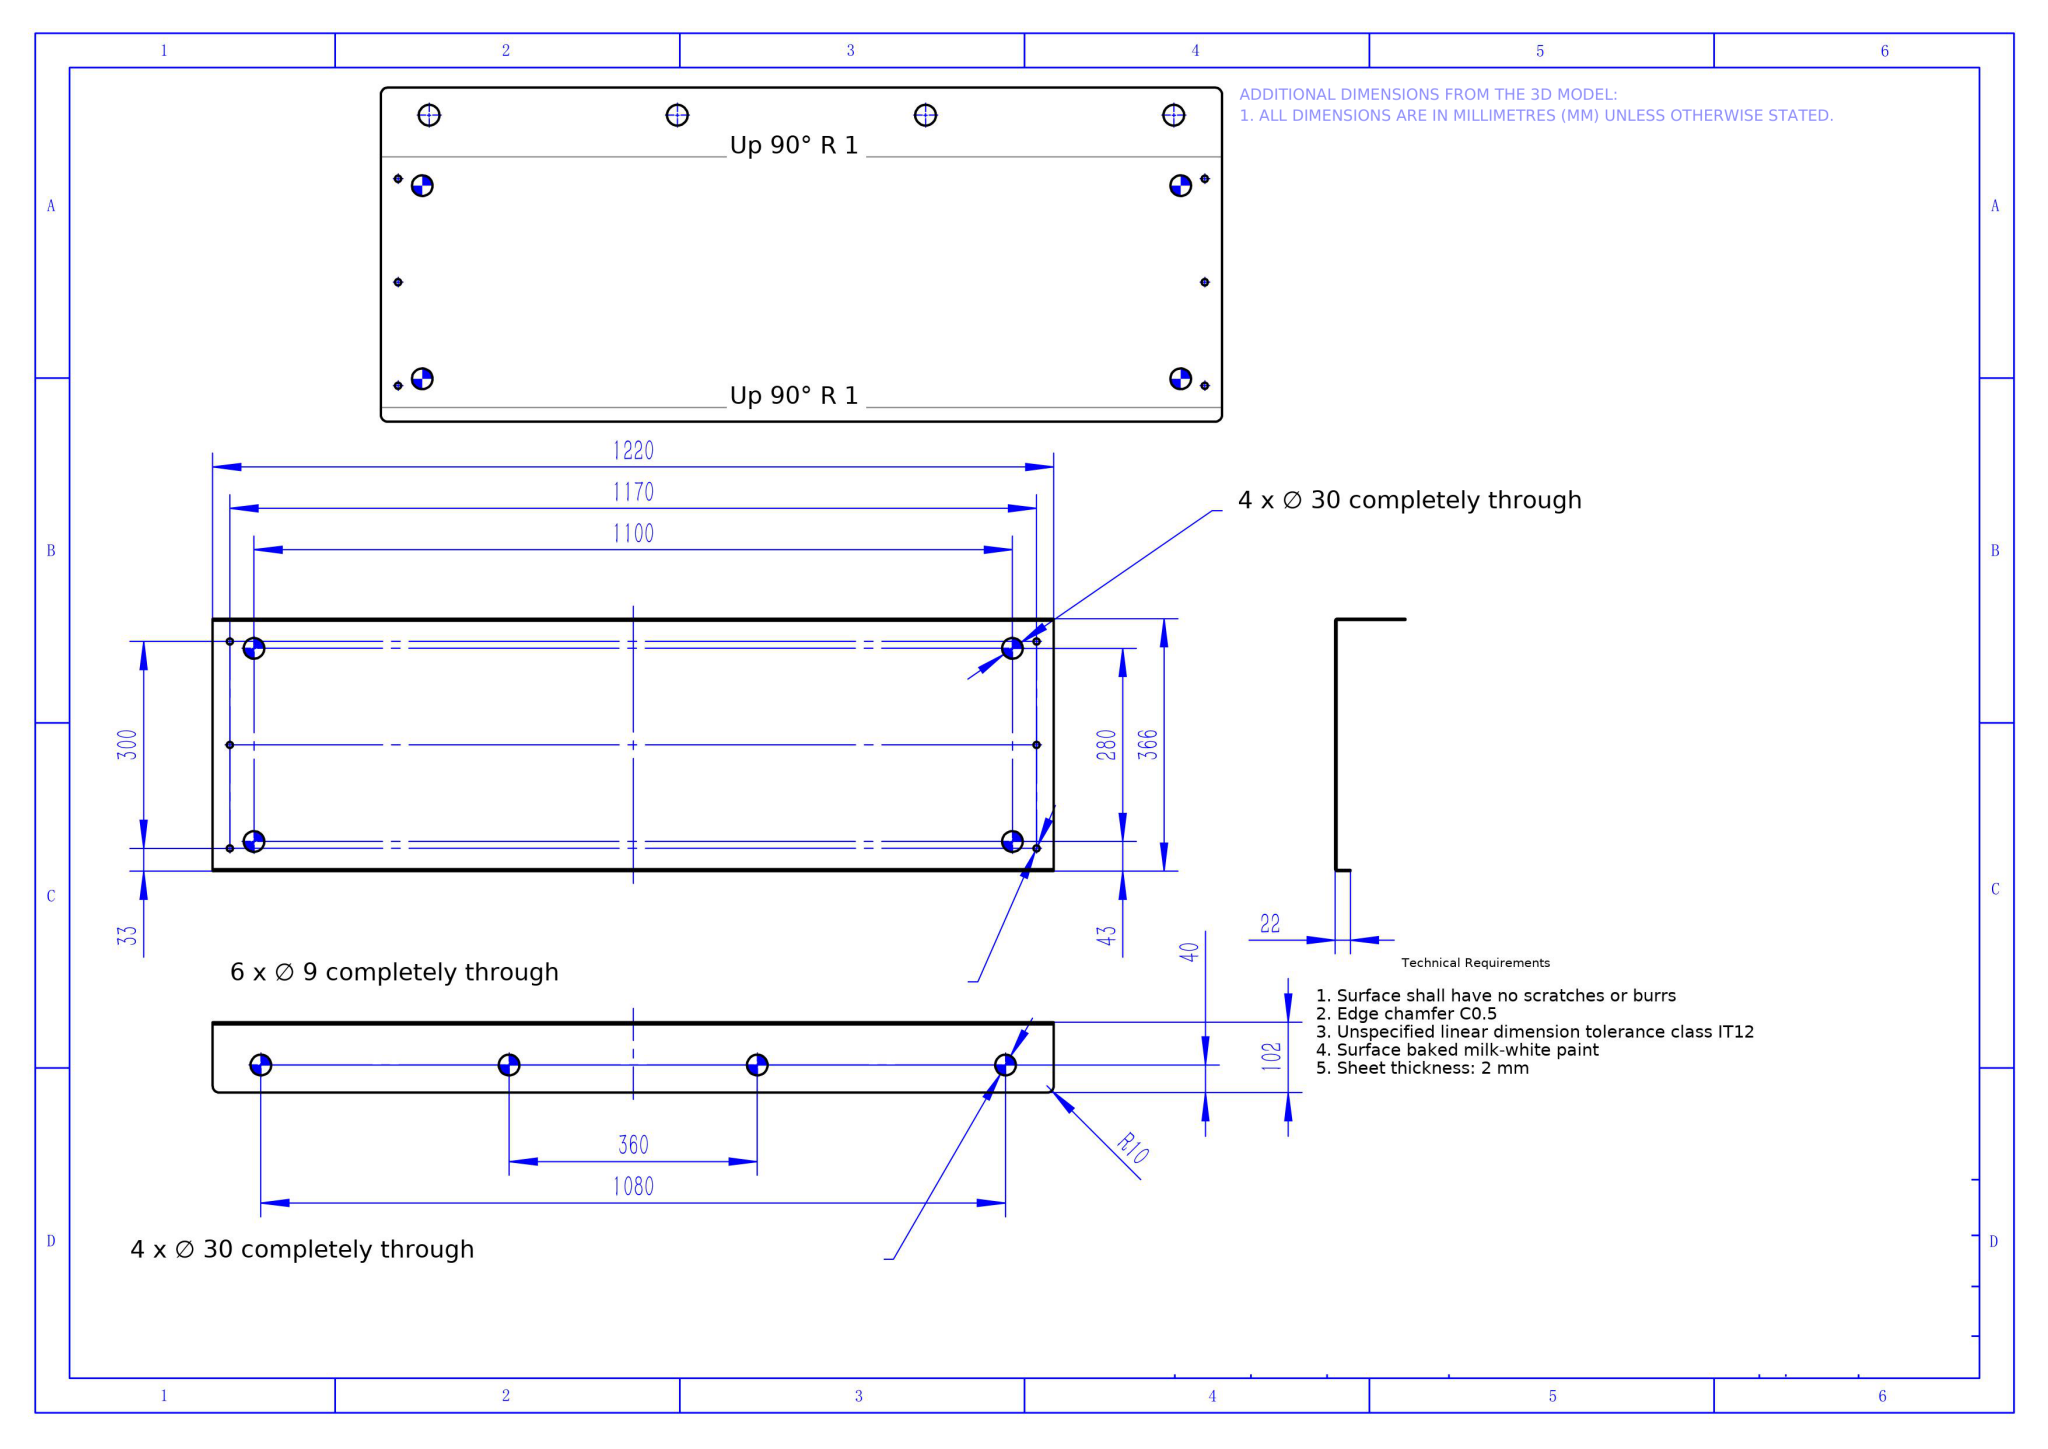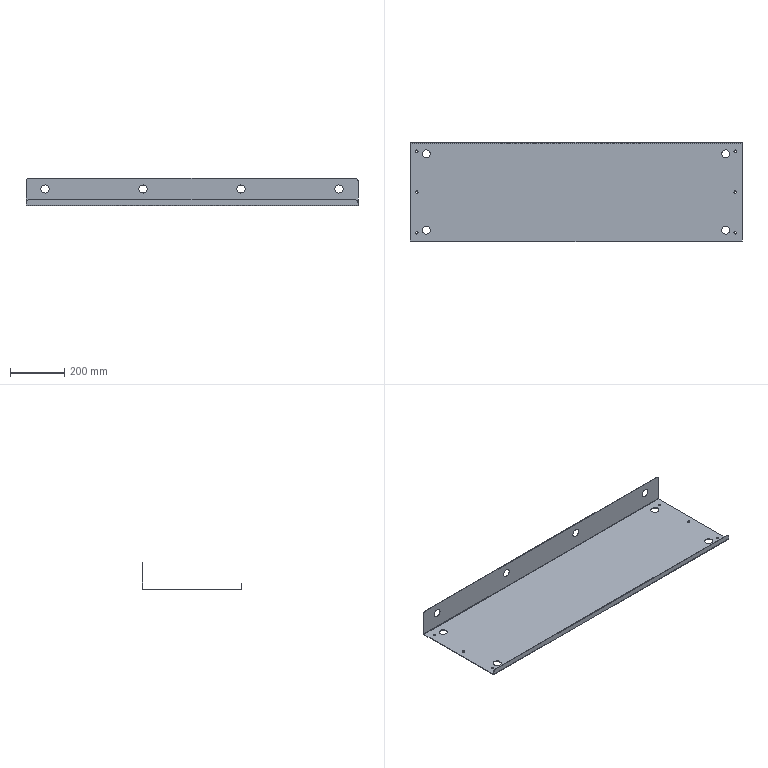Part | NX | mm | Elongated U-Channel Mounting Bracket With Dual End Tabs | 1 solid | 54 faces | box 1220 x 366 x 102 mm | volume 1169406 mm3 | cylinder 36 | plane 18 | commonest cylinder face diameters 30 x16 9 x12 20 x4 6 x2 2 x2